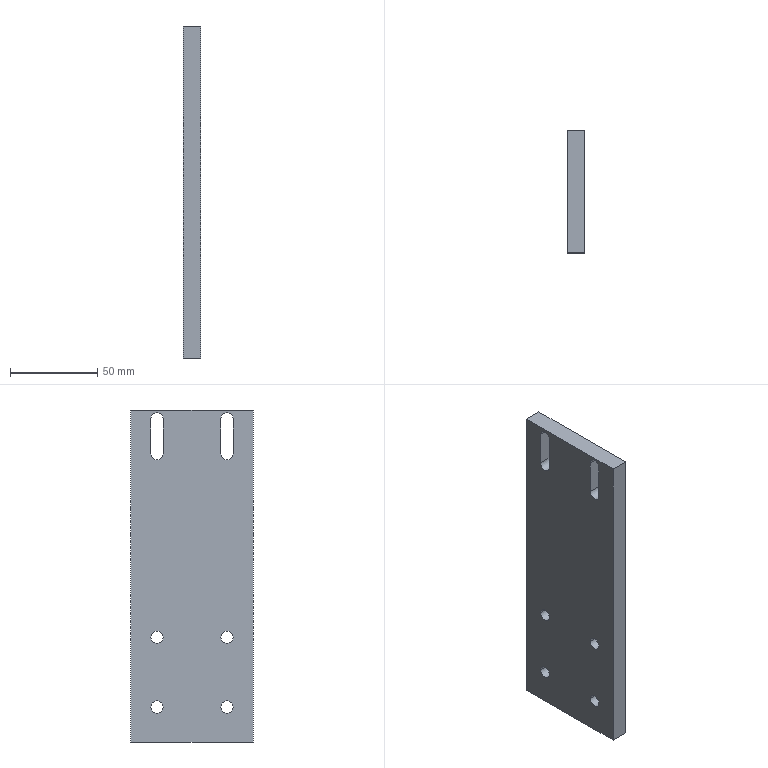Component | SolidWorks | 30-71A-1 | 1 solid | 22 faces | box 10 x 70 x 190 mm | volume 127891 mm3 | cylinder 12 | plane 10 | commonest cylinder face diameters 7 x12
build123d program:
from build123d import *

# Parameters (mm, degrees)
SKETCH1_W          = 70
SKETCH1_H          = 190
EXTRUDE1_DEPTH     = 10
SKETCH8_R          = 3.5
CUT_EXTRUDE1_DEPTH = 102.735
CUT_EXTRUDE2_DEPTH = 10


with BuildPart() as part:
    # Sketch1 → Extrude1 (new body)
    with BuildSketch(Plane.XY):
        Rectangle(SKETCH1_W, SKETCH1_H)
    extrude(amount=EXTRUDE1_DEPTH)

    # Sketch8 → Cut-Extrude1 (cut, through all)
    with BuildSketch(Plane(origin=(0, 0, 0), x_dir=(-1, 0, 0), z_dir=(0, 0, -1))):
        with Locations((-20, -75)):
            Circle(SKETCH8_R)
        with Locations(Location((20, -75, 0), (0, 0, 180))):
            Circle(SKETCH8_R)
        with Locations((20, -35)):
            Circle(SKETCH8_R)
        with Locations(Location((-20, -35, 0), (0, 0, 180))):
            Circle(SKETCH8_R)
    extrude(amount=-CUT_EXTRUDE1_DEPTH, mode=Mode.SUBTRACT)

    # Sketch11 → Cut-Extrude2 (cut)
    with BuildSketch(Plane(origin=(0, 0, 0), x_dir=(-1, 0, 0), z_dir=(0, 0, -1))):
        with BuildLine():
            Line((-23.5, 90), (-23.5, 70))
            ThreePointArc((-23.5, 70), (-20, 66.5), (-16.5, 70))
            Line((-16.5, 70), (-16.5, 90))
            ThreePointArc((-16.5, 90), (-20, 93.5), (-23.5, 90))
        make_face()
        with BuildLine():
            Line((16.5, 70), (16.5, 90))
            ThreePointArc((16.5, 90), (20, 93.5), (23.5, 90))
            Line((23.5, 90), (23.5, 70))
            ThreePointArc((23.5, 70), (20, 66.5), (16.5, 70))
        make_face()
    extrude(amount=-CUT_EXTRUDE2_DEPTH, mode=Mode.SUBTRACT)


solid = part.part

# Placed as in the assembly
solid = solid.moved(Location((302.57, -515.845, 55), (90, -90, 0)))
STEP:
#1=COLOUR_RGB('',0.7922,0.8196,0.9333);
#2=FILL_AREA_STYLE_COLOUR('',#1);
#3=FILL_AREA_STYLE('',(#2));
#4=SURFACE_STYLE_FILL_AREA(#3);
#5=SURFACE_SIDE_STYLE('',(#4));
#6=SURFACE_STYLE_USAGE(.BOTH.,#5);
#7=PRESENTATION_STYLE_ASSIGNMENT((#6));
#8=CARTESIAN_POINT('',(11.519,-21.234,0.7874));
#9=VERTEX_POINT('',#8);
#10=CARTESIAN_POINT('',(11.519,-20.958,0.7874));
#11=VERTEX_POINT('',#10);
#12=CARTESIAN_POINT('',(11.519,-21.096,0.7874));
#13=DIRECTION('',(1.,0.,0.));
#14=DIRECTION('',(0.,-1.,0.));
#15=AXIS2_PLACEMENT_3D('',#12,#13,#14);
#16=CIRCLE('',#15,0.1378);
#17=EDGE_CURVE('',#9,#11,#16,.T.);
#18=ORIENTED_EDGE('',*,*,#17,.F.);
#19=CARTESIAN_POINT('',(11.912,-21.234,0.7874));
#20=VERTEX_POINT('',#19);
#21=CARTESIAN_POINT('',(11.519,-21.234,0.7874));
#22=DIRECTION('',(1.,0.,0.));
#23=VECTOR('',#22,39.37);
#24=LINE('',#21,#23);
#25=EDGE_CURVE('',#9,#20,#24,.T.);
#26=ORIENTED_EDGE('',*,*,#25,.T.);
#27=CARTESIAN_POINT('',(11.912,-20.958,0.7874));
#28=VERTEX_POINT('',#27);
#29=CARTESIAN_POINT('',(11.912,-21.096,0.7874));
#30=DIRECTION('',(1.,0.,0.));
#31=DIRECTION('',(0.,-1.,0.));
#32=AXIS2_PLACEMENT_3D('',#29,#30,#31);
#33=CIRCLE('',#32,0.1378);
#34=EDGE_CURVE('',#20,#28,#33,.T.);
#35=ORIENTED_EDGE('',*,*,#34,.T.);
#36=CARTESIAN_POINT('',(11.519,-20.958,0.7874));
#37=DIRECTION('',(1.,0.,0.));
#38=VECTOR('',#37,39.37);
#39=LINE('',#36,#38);
#40=EDGE_CURVE('',#11,#28,#39,.T.);
#41=ORIENTED_EDGE('',*,*,#40,.F.);
#42=EDGE_LOOP('',(#18,#26,#35,#41));
#43=FACE_OUTER_BOUND('',#42,.T.);
#44=CARTESIAN_POINT('',(11.519,-21.096,0.7874));
#45=DIRECTION('',(1.,0.,0.));
#46=DIRECTION('',(0.,1.,0.));
#47=AXIS2_PLACEMENT_3D('',#44,#45,#46);
#48=CYLINDRICAL_SURFACE('',#47,0.1378);
#49=ADVANCED_FACE('',(#43),#48,.F.);
#50=CARTESIAN_POINT('',(11.519,-19.659,0.7874));
#51=VERTEX_POINT('',#50);
#52=CARTESIAN_POINT('',(11.519,-19.384,0.7874));
#53=VERTEX_POINT('',#52);
#54=CARTESIAN_POINT('',(11.519,-19.521,0.7874));
#55=DIRECTION('',(1.,0.,0.));
#56=DIRECTION('',(0.,1.,0.));
#57=AXIS2_PLACEMENT_3D('',#54,#55,#56);
#58=CIRCLE('',#57,0.1378);
#59=EDGE_CURVE('',#51,#53,#58,.T.);
#60=ORIENTED_EDGE('',*,*,#59,.F.);
#61=CARTESIAN_POINT('',(11.912,-19.659,0.7874));
#62=VERTEX_POINT('',#61);
#63=CARTESIAN_POINT('',(11.519,-19.659,0.7874));
#64=DIRECTION('',(1.,0.,0.));
#65=VECTOR('',#64,39.37);
#66=LINE('',#63,#65);
#67=EDGE_CURVE('',#51,#62,#66,.T.);
#68=ORIENTED_EDGE('',*,*,#67,.T.);
#69=CARTESIAN_POINT('',(11.912,-19.384,0.7874));
#70=VERTEX_POINT('',#69);
#71=CARTESIAN_POINT('',(11.912,-19.521,0.7874));
#72=DIRECTION('',(1.,0.,0.));
#73=DIRECTION('',(0.,1.,0.));
#74=AXIS2_PLACEMENT_3D('',#71,#72,#73);
#75=CIRCLE('',#74,0.1378);
#76=EDGE_CURVE('',#62,#70,#75,.T.);
#77=ORIENTED_EDGE('',*,*,#76,.T.);
#78=CARTESIAN_POINT('',(11.519,-19.384,0.7874));
#79=DIRECTION('',(1.,0.,0.));
#80=VECTOR('',#79,39.37);
#81=LINE('',#78,#80);
#82=EDGE_CURVE('',#53,#70,#81,.T.);
#83=ORIENTED_EDGE('',*,*,#82,.F.);
#84=EDGE_LOOP('',(#60,#68,#77,#83));
#85=FACE_OUTER_BOUND('',#84,.T.);
#86=CARTESIAN_POINT('',(11.519,-19.521,0.7874));
#87=DIRECTION('',(1.,0.,0.));
#88=DIRECTION('',(0.,1.,0.));
#89=AXIS2_PLACEMENT_3D('',#86,#87,#88);
#90=CYLINDRICAL_SURFACE('',#89,0.1378);
#91=ADVANCED_FACE('',(#85),#90,.F.);
#92=CARTESIAN_POINT('',(11.519,-19.659,-0.7874));
#93=VERTEX_POINT('',#92);
#94=CARTESIAN_POINT('',(11.519,-19.384,-0.7874));
#95=VERTEX_POINT('',#94);
#96=CARTESIAN_POINT('',(11.519,-19.521,-0.7874));
#97=DIRECTION('',(1.,0.,0.));
#98=DIRECTION('',(0.,-1.,0.));
#99=AXIS2_PLACEMENT_3D('',#96,#97,#98);
#100=CIRCLE('',#99,0.1378);
#101=EDGE_CURVE('',#93,#95,#100,.T.);
#102=ORIENTED_EDGE('',*,*,#101,.F.);
#103=CARTESIAN_POINT('',(11.912,-19.659,-0.7874));
#104=VERTEX_POINT('',#103);
#105=CARTESIAN_POINT('',(11.519,-19.659,-0.7874));
#106=DIRECTION('',(1.,0.,0.));
#107=VECTOR('',#106,39.37);
#108=LINE('',#105,#107);
#109=EDGE_CURVE('',#93,#104,#108,.T.);
#110=ORIENTED_EDGE('',*,*,#109,.T.);
#111=CARTESIAN_POINT('',(11.912,-19.384,-0.7874));
#112=VERTEX_POINT('',#111);
#113=CARTESIAN_POINT('',(11.912,-19.521,-0.7874));
#114=DIRECTION('',(1.,0.,0.));
#115=DIRECTION('',(0.,-1.,0.));
#116=AXIS2_PLACEMENT_3D('',#113,#114,#115);
#117=CIRCLE('',#116,0.1378);
#118=EDGE_CURVE('',#104,#112,#117,.T.);
#119=ORIENTED_EDGE('',*,*,#118,.T.);
#120=CARTESIAN_POINT('',(11.519,-19.384,-0.7874));
#121=DIRECTION('',(1.,0.,0.));
#122=VECTOR('',#121,39.37);
#123=LINE('',#120,#122);
#124=EDGE_CURVE('',#95,#112,#123,.T.);
#125=ORIENTED_EDGE('',*,*,#124,.F.);
#126=EDGE_LOOP('',(#102,#110,#119,#125));
#127=FACE_OUTER_BOUND('',#126,.T.);
#128=CARTESIAN_POINT('',(11.519,-19.521,-0.7874));
#129=DIRECTION('',(1.,0.,0.));
#130=DIRECTION('',(0.,1.,0.));
#131=AXIS2_PLACEMENT_3D('',#128,#129,#130);
#132=CYLINDRICAL_SURFACE('',#131,0.1378);
#133=ADVANCED_FACE('',(#127),#132,.F.);
#134=CARTESIAN_POINT('',(11.519,-21.234,-0.7874));
#135=VERTEX_POINT('',#134);
#136=CARTESIAN_POINT('',(11.519,-20.958,-0.7874));
#137=VERTEX_POINT('',#136);
#138=CARTESIAN_POINT('',(11.519,-21.096,-0.7874));
#139=DIRECTION('',(1.,0.,0.));
#140=DIRECTION('',(0.,1.,0.));
#141=AXIS2_PLACEMENT_3D('',#138,#139,#140);
#142=CIRCLE('',#141,0.1378);
#143=EDGE_CURVE('',#135,#137,#142,.T.);
#144=ORIENTED_EDGE('',*,*,#143,.F.);
#145=CARTESIAN_POINT('',(11.912,-21.234,-0.7874));
#146=VERTEX_POINT('',#145);
#147=CARTESIAN_POINT('',(11.519,-21.234,-0.7874));
#148=DIRECTION('',(1.,0.,0.));
#149=VECTOR('',#148,39.37);
#150=LINE('',#147,#149);
#151=EDGE_CURVE('',#135,#146,#150,.T.);
#152=ORIENTED_EDGE('',*,*,#151,.T.);
#153=CARTESIAN_POINT('',(11.912,-20.958,-0.7874));
#154=VERTEX_POINT('',#153);
#155=CARTESIAN_POINT('',(11.912,-21.096,-0.7874));
#156=DIRECTION('',(1.,0.,0.));
#157=DIRECTION('',(0.,1.,0.));
#158=AXIS2_PLACEMENT_3D('',#155,#156,#157);
#159=CIRCLE('',#158,0.1378);
#160=EDGE_CURVE('',#146,#154,#159,.T.);
#161=ORIENTED_EDGE('',*,*,#160,.T.);
#162=CARTESIAN_POINT('',(11.519,-20.958,-0.7874));
#163=DIRECTION('',(1.,0.,0.));
#164=VECTOR('',#163,39.37);
#165=LINE('',#162,#164);
#166=EDGE_CURVE('',#137,#154,#165,.T.);
#167=ORIENTED_EDGE('',*,*,#166,.F.);
#168=EDGE_LOOP('',(#144,#152,#161,#167));
#169=FACE_OUTER_BOUND('',#168,.T.);
#170=CARTESIAN_POINT('',(11.519,-21.096,-0.7874));
#171=DIRECTION('',(1.,0.,0.));
#172=DIRECTION('',(0.,1.,0.));
#173=AXIS2_PLACEMENT_3D('',#170,#171,#172);
#174=CYLINDRICAL_SURFACE('',#173,0.1378);
#175=ADVANCED_FACE('',(#169),#174,.F.);
#176=CARTESIAN_POINT('',(11.912,-18.931,5.906));
#177=VERTEX_POINT('',#176);
#178=CARTESIAN_POINT('',(11.912,-18.931,-1.575));
#179=VERTEX_POINT('',#178);
#180=CARTESIAN_POINT('',(11.912,-18.931,5.906));
#181=DIRECTION('',(0.,0.,-1.));
#182=VECTOR('',#181,39.37);
#183=LINE('',#180,#182);
#184=EDGE_CURVE('',#177,#179,#183,.T.);
#185=ORIENTED_EDGE('',*,*,#184,.T.);
#186=CARTESIAN_POINT('',(11.519,-18.931,-1.575));
#187=VERTEX_POINT('',#186);
#188=CARTESIAN_POINT('',(11.519,-18.931,-1.575));
#189=DIRECTION('',(1.,0.,0.));
#190=VECTOR('',#189,39.37);
#191=LINE('',#188,#190);
#192=EDGE_CURVE('',#187,#179,#191,.T.);
#193=ORIENTED_EDGE('',*,*,#192,.F.);
#194=CARTESIAN_POINT('',(11.519,-18.931,5.906));
#195=VERTEX_POINT('',#194);
#196=CARTESIAN_POINT('',(11.519,-18.931,5.906));
#197=DIRECTION('',(0.,0.,-1.));
#198=VECTOR('',#197,39.37);
#199=LINE('',#196,#198);
#200=EDGE_CURVE('',#195,#187,#199,.T.);
#201=ORIENTED_EDGE('',*,*,#200,.F.);
#202=CARTESIAN_POINT('',(11.519,-18.931,5.906));
#203=DIRECTION('',(1.,0.,0.));
#204=VECTOR('',#203,39.37);
#205=LINE('',#202,#204);
#206=EDGE_CURVE('',#195,#177,#205,.T.);
#207=ORIENTED_EDGE('',*,*,#206,.T.);
#208=EDGE_LOOP('',(#185,#193,#201,#207));
#209=FACE_OUTER_BOUND('',#208,.T.);
#210=CARTESIAN_POINT('',(11.519,-18.931,5.906));
#211=DIRECTION('',(0.,-1.,0.));
#212=DIRECTION('',(1.,0.,0.));
#213=AXIS2_PLACEMENT_3D('',#210,#211,#212);
#214=PLANE('',#213);
#215=ADVANCED_FACE('',(#209),#214,.F.);
#216=CARTESIAN_POINT('',(11.912,-21.687,-1.575));
#217=VERTEX_POINT('',#216);
#218=CARTESIAN_POINT('',(11.912,-18.931,-1.575));
#219=DIRECTION('',(-0.,-1.,0.));
#220=VECTOR('',#219,39.37);
#221=LINE('',#218,#220);
#222=EDGE_CURVE('',#179,#217,#221,.T.);
#223=ORIENTED_EDGE('',*,*,#222,.T.);
#224=CARTESIAN_POINT('',(11.519,-21.687,-1.575));
#225=VERTEX_POINT('',#224);
#226=CARTESIAN_POINT('',(11.519,-21.687,-1.575));
#227=DIRECTION('',(1.,0.,0.));
#228=VECTOR('',#227,39.37);
#229=LINE('',#226,#228);
#230=EDGE_CURVE('',#225,#217,#229,.T.);
#231=ORIENTED_EDGE('',*,*,#230,.F.);
#232=CARTESIAN_POINT('',(11.519,-18.931,-1.575));
#233=DIRECTION('',(-0.,-1.,0.));
#234=VECTOR('',#233,39.37);
#235=LINE('',#232,#234);
#236=EDGE_CURVE('',#187,#225,#235,.T.);
#237=ORIENTED_EDGE('',*,*,#236,.F.);
#238=ORIENTED_EDGE('',*,*,#192,.T.);
#239=EDGE_LOOP('',(#223,#231,#237,#238));
#240=FACE_OUTER_BOUND('',#239,.T.);
#241=CARTESIAN_POINT('',(11.519,-18.931,-1.575));
#242=DIRECTION('',(-0.,0.,1.));
#243=DIRECTION('',(-1.,-0.,-0.));
#244=AXIS2_PLACEMENT_3D('',#241,#242,#243);
#245=PLANE('',#244);
#246=ADVANCED_FACE('',(#240),#245,.F.);
#247=CARTESIAN_POINT('',(11.912,-21.687,5.906));
#248=VERTEX_POINT('',#247);
#249=CARTESIAN_POINT('',(11.912,-21.687,5.906));
#250=DIRECTION('',(-0.,0.,1.));
#251=VECTOR('',#250,39.37);
#252=LINE('',#249,#251);
#253=EDGE_CURVE('',#217,#248,#252,.T.);
#254=ORIENTED_EDGE('',*,*,#253,.T.);
#255=CARTESIAN_POINT('',(11.519,-21.687,5.906));
#256=VERTEX_POINT('',#255);
#257=CARTESIAN_POINT('',(11.519,-21.687,5.906));
#258=DIRECTION('',(1.,0.,0.));
#259=VECTOR('',#258,39.37);
#260=LINE('',#257,#259);
#261=EDGE_CURVE('',#256,#248,#260,.T.);
#262=ORIENTED_EDGE('',*,*,#261,.F.);
#263=CARTESIAN_POINT('',(11.519,-21.687,5.906));
#264=DIRECTION('',(-0.,0.,1.));
#265=VECTOR('',#264,39.37);
#266=LINE('',#263,#265);
#267=EDGE_CURVE('',#225,#256,#266,.T.);
#268=ORIENTED_EDGE('',*,*,#267,.F.);
#269=ORIENTED_EDGE('',*,*,#230,.T.);
#270=EDGE_LOOP('',(#254,#262,#268,#269));
#271=FACE_OUTER_BOUND('',#270,.T.);
#272=CARTESIAN_POINT('',(11.519,-21.687,5.906));
#273=DIRECTION('',(-0.,1.,-0.));
#274=DIRECTION('',(-1.,-0.,-0.));
#275=AXIS2_PLACEMENT_3D('',#272,#273,#274);
#276=PLANE('',#275);
#277=ADVANCED_FACE('',(#271),#276,.F.);
#278=CARTESIAN_POINT('',(11.912,-18.931,5.906));
#279=DIRECTION('',(0.,1.,-0.));
#280=VECTOR('',#279,39.37);
#281=LINE('',#278,#280);
#282=EDGE_CURVE('',#248,#177,#281,.T.);
#283=ORIENTED_EDGE('',*,*,#282,.T.);
#284=ORIENTED_EDGE('',*,*,#206,.F.);
#285=CARTESIAN_POINT('',(11.519,-18.931,5.906));
#286=DIRECTION('',(0.,1.,-0.));
#287=VECTOR('',#286,39.37);
#288=LINE('',#285,#287);
#289=EDGE_CURVE('',#256,#195,#288,.T.);
#290=ORIENTED_EDGE('',*,*,#289,.F.);
#291=ORIENTED_EDGE('',*,*,#261,.T.);
#292=EDGE_LOOP('',(#283,#284,#290,#291));
#293=FACE_OUTER_BOUND('',#292,.T.);
#294=CARTESIAN_POINT('',(11.519,-18.931,5.906));
#295=DIRECTION('',(0.,-0.,-1.));
#296=DIRECTION('',(1.,0.,0.));
#297=AXIS2_PLACEMENT_3D('',#294,#295,#296);
#298=PLANE('',#297);
#299=ADVANCED_FACE('',(#293),#298,.F.);
#300=CARTESIAN_POINT('',(11.519,-20.958,5.709));
#301=VERTEX_POINT('',#300);
#302=CARTESIAN_POINT('',(11.519,-21.234,5.709));
#303=VERTEX_POINT('',#302);
#304=CARTESIAN_POINT('',(11.519,-21.096,5.709));
#305=DIRECTION('',(1.,0.,0.));
#306=DIRECTION('',(0.,1.,0.));
#307=AXIS2_PLACEMENT_3D('',#304,#305,#306);
#308=CIRCLE('',#307,0.1378);
#309=EDGE_CURVE('',#301,#303,#308,.T.);
#310=ORIENTED_EDGE('',*,*,#309,.T.);
#311=CARTESIAN_POINT('',(11.519,-21.234,4.921));
#312=VERTEX_POINT('',#311);
#313=CARTESIAN_POINT('',(11.519,-21.234,5.709));
#314=DIRECTION('',(0.,0.,-1.));
#315=VECTOR('',#314,39.37);
#316=LINE('',#313,#315);
#317=EDGE_CURVE('',#303,#312,#316,.T.);
#318=ORIENTED_EDGE('',*,*,#317,.T.);
#319=CARTESIAN_POINT('',(11.519,-20.958,4.921));
#320=VERTEX_POINT('',#319);
#321=CARTESIAN_POINT('',(11.519,-21.096,4.921));
#322=DIRECTION('',(1.,0.,0.));
#323=DIRECTION('',(0.,1.,0.));
#324=AXIS2_PLACEMENT_3D('',#321,#322,#323);
#325=CIRCLE('',#324,0.1378);
#326=EDGE_CURVE('',#312,#320,#325,.T.);
#327=ORIENTED_EDGE('',*,*,#326,.T.);
#328=CARTESIAN_POINT('',(11.519,-20.958,4.921));
#329=DIRECTION('',(-0.,0.,1.));
#330=VECTOR('',#329,39.37);
#331=LINE('',#328,#330);
#332=EDGE_CURVE('',#320,#301,#331,.T.);
#333=ORIENTED_EDGE('',*,*,#332,.T.);
#334=EDGE_LOOP('',(#310,#318,#327,#333));
#335=FACE_BOUND('',#334,.T.);
#336=CARTESIAN_POINT('',(11.519,-19.659,4.921));
#337=VERTEX_POINT('',#336);
#338=CARTESIAN_POINT('',(11.519,-19.384,4.921));
#339=VERTEX_POINT('',#338);
#340=CARTESIAN_POINT('',(11.519,-19.521,4.921));
#341=DIRECTION('',(1.,0.,0.));
#342=DIRECTION('',(0.,-1.,0.));
#343=AXIS2_PLACEMENT_3D('',#340,#341,#342);
#344=CIRCLE('',#343,0.1378);
#345=EDGE_CURVE('',#337,#339,#344,.T.);
#346=ORIENTED_EDGE('',*,*,#345,.T.);
#347=CARTESIAN_POINT('',(11.519,-19.384,5.709));
#348=VERTEX_POINT('',#347);
#349=CARTESIAN_POINT('',(11.519,-19.384,5.709));
#350=DIRECTION('',(-0.,0.,1.));
#351=VECTOR('',#350,39.37);
#352=LINE('',#349,#351);
#353=EDGE_CURVE('',#339,#348,#352,.T.);
#354=ORIENTED_EDGE('',*,*,#353,.T.);
#355=CARTESIAN_POINT('',(11.519,-19.659,5.709));
#356=VERTEX_POINT('',#355);
#357=CARTESIAN_POINT('',(11.519,-19.521,5.709));
#358=DIRECTION('',(1.,0.,0.));
#359=DIRECTION('',(0.,-1.,0.));
#360=AXIS2_PLACEMENT_3D('',#357,#358,#359);
#361=CIRCLE('',#360,0.1378);
#362=EDGE_CURVE('',#348,#356,#361,.T.);
#363=ORIENTED_EDGE('',*,*,#362,.T.);
#364=CARTESIAN_POINT('',(11.519,-19.659,4.921));
#365=DIRECTION('',(0.,0.,-1.));
#366=VECTOR('',#365,39.37);
#367=LINE('',#364,#366);
#368=EDGE_CURVE('',#356,#337,#367,.T.);
#369=ORIENTED_EDGE('',*,*,#368,.T.);
#370=EDGE_LOOP('',(#346,#354,#363,#369));
#371=FACE_BOUND('',#370,.T.);
#372=CARTESIAN_POINT('',(11.519,-21.096,0.7874));
#373=DIRECTION('',(1.,0.,0.));
#374=DIRECTION('',(0.,-1.,0.));
#375=AXIS2_PLACEMENT_3D('',#372,#373,#374);
#376=CIRCLE('',#375,0.1378);
#377=EDGE_CURVE('',#11,#9,#376,.T.);
#378=ORIENTED_EDGE('',*,*,#377,.T.);
#379=ORIENTED_EDGE('',*,*,#17,.T.);
#380=EDGE_LOOP('',(#378,#379));
#381=FACE_BOUND('',#380,.T.);
#382=CARTESIAN_POINT('',(11.519,-19.521,0.7874));
#383=DIRECTION('',(1.,0.,0.));
#384=DIRECTION('',(0.,1.,0.));
#385=AXIS2_PLACEMENT_3D('',#382,#383,#384);
#386=CIRCLE('',#385,0.1378);
#387=EDGE_CURVE('',#53,#51,#386,.T.);
#388=ORIENTED_EDGE('',*,*,#387,.T.);
#389=ORIENTED_EDGE('',*,*,#59,.T.);
#390=EDGE_LOOP('',(#388,#389));
#391=FACE_BOUND('',#390,.T.);
#392=CARTESIAN_POINT('',(11.519,-19.521,-0.7874));
#393=DIRECTION('',(1.,0.,0.));
#394=DIRECTION('',(0.,-1.,0.));
#395=AXIS2_PLACEMENT_3D('',#392,#393,#394);
#396=CIRCLE('',#395,0.1378);
#397=EDGE_CURVE('',#95,#93,#396,.T.);
#398=ORIENTED_EDGE('',*,*,#397,.T.);
#399=ORIENTED_EDGE('',*,*,#101,.T.);
#400=EDGE_LOOP('',(#398,#399));
#401=FACE_BOUND('',#400,.T.);
#402=CARTESIAN_POINT('',(11.519,-21.096,-0.7874));
#403=DIRECTION('',(1.,0.,0.));
#404=DIRECTION('',(0.,1.,0.));
#405=AXIS2_PLACEMENT_3D('',#402,#403,#404);
#406=CIRCLE('',#405,0.1378);
#407=EDGE_CURVE('',#137,#135,#406,.T.);
#408=ORIENTED_EDGE('',*,*,#407,.T.);
#409=ORIENTED_EDGE('',*,*,#143,.T.);
#410=EDGE_LOOP('',(#408,#409));
#411=FACE_BOUND('',#410,.T.);
#412=ORIENTED_EDGE('',*,*,#200,.T.);
#413=ORIENTED_EDGE('',*,*,#236,.T.);
#414=ORIENTED_EDGE('',*,*,#267,.T.);
#415=ORIENTED_EDGE('',*,*,#289,.T.);
#416=EDGE_LOOP('',(#412,#413,#414,#415));
#417=FACE_OUTER_BOUND('',#416,.T.);
#418=CARTESIAN_POINT('',(11.519,-18.931,-1.575));
#419=DIRECTION('',(-1.,0.,-0.));
#420=DIRECTION('',(-0.,-1.,0.));
#421=AXIS2_PLACEMENT_3D('',#418,#419,#420);
#422=PLANE('',#421);
#423=ADVANCED_FACE('',(#335,#371,#381,#391,#401,#411,#417),#422,.T.);
#424=CARTESIAN_POINT('',(11.912,-21.234,5.709));
#425=VERTEX_POINT('',#424);
#426=CARTESIAN_POINT('',(11.912,-21.234,4.921));
#427=VERTEX_POINT('',#426);
#428=CARTESIAN_POINT('',(11.912,-21.234,5.709));
#429=DIRECTION('',(0.,0.,-1.));
#430=VECTOR('',#429,39.37);
#431=LINE('',#428,#430);
#432=EDGE_CURVE('',#425,#427,#431,.T.);
#433=ORIENTED_EDGE('',*,*,#432,.F.);
#434=CARTESIAN_POINT('',(11.912,-20.958,5.709));
#435=VERTEX_POINT('',#434);
#436=CARTESIAN_POINT('',(11.912,-21.096,5.709));
#437=DIRECTION('',(1.,0.,0.));
#438=DIRECTION('',(0.,1.,0.));
#439=AXIS2_PLACEMENT_3D('',#436,#437,#438);
#440=CIRCLE('',#439,0.1378);
#441=EDGE_CURVE('',#435,#425,#440,.T.);
#442=ORIENTED_EDGE('',*,*,#441,.F.);
#443=CARTESIAN_POINT('',(11.912,-20.958,4.921));
#444=VERTEX_POINT('',#443);
#445=CARTESIAN_POINT('',(11.912,-20.958,4.921));
#446=DIRECTION('',(-0.,0.,1.));
#447=VECTOR('',#446,39.37);
#448=LINE('',#445,#447);
#449=EDGE_CURVE('',#444,#435,#448,.T.);
#450=ORIENTED_EDGE('',*,*,#449,.F.);
#451=CARTESIAN_POINT('',(11.912,-21.096,4.921));
#452=DIRECTION('',(1.,0.,0.));
#453=DIRECTION('',(0.,1.,0.));
#454=AXIS2_PLACEMENT_3D('',#451,#452,#453);
#455=CIRCLE('',#454,0.1378);
#456=EDGE_CURVE('',#427,#444,#455,.T.);
#457=ORIENTED_EDGE('',*,*,#456,.F.);
#458=EDGE_LOOP('',(#433,#442,#450,#457));
#459=FACE_BOUND('',#458,.T.);
#460=CARTESIAN_POINT('',(11.912,-19.384,4.921));
#461=VERTEX_POINT('',#460);
#462=CARTESIAN_POINT('',(11.912,-19.384,5.709));
#463=VERTEX_POINT('',#462);
#464=CARTESIAN_POINT('',(11.912,-19.384,5.709));
#465=DIRECTION('',(-0.,0.,1.));
#466=VECTOR('',#465,39.37);
#467=LINE('',#464,#466);
#468=EDGE_CURVE('',#461,#463,#467,.T.);
#469=ORIENTED_EDGE('',*,*,#468,.F.);
#470=CARTESIAN_POINT('',(11.912,-19.659,4.921));
#471=VERTEX_POINT('',#470);
#472=CARTESIAN_POINT('',(11.912,-19.521,4.921));
#473=DIRECTION('',(1.,0.,0.));
#474=DIRECTION('',(0.,-1.,0.));
#475=AXIS2_PLACEMENT_3D('',#472,#473,#474);
#476=CIRCLE('',#475,0.1378);
#477=EDGE_CURVE('',#471,#461,#476,.T.);
#478=ORIENTED_EDGE('',*,*,#477,.F.);
#479=CARTESIAN_POINT('',(11.912,-19.659,5.709));
#480=VERTEX_POINT('',#479);
#481=CARTESIAN_POINT('',(11.912,-19.659,4.921));
#482=DIRECTION('',(0.,0.,-1.));
#483=VECTOR('',#482,39.37);
#484=LINE('',#481,#483);
#485=EDGE_CURVE('',#480,#471,#484,.T.);
#486=ORIENTED_EDGE('',*,*,#485,.F.);
#487=CARTESIAN_POINT('',(11.912,-19.521,5.709));
#488=DIRECTION('',(1.,0.,0.));
#489=DIRECTION('',(0.,-1.,0.));
#490=AXIS2_PLACEMENT_3D('',#487,#488,#489);
#491=CIRCLE('',#490,0.1378);
#492=EDGE_CURVE('',#463,#480,#491,.T.);
#493=ORIENTED_EDGE('',*,*,#492,.F.);
#494=EDGE_LOOP('',(#469,#478,#486,#493));
#495=FACE_BOUND('',#494,.T.);
#496=CARTESIAN_POINT('',(11.912,-21.096,0.7874));
#497=DIRECTION('',(1.,0.,0.));
#498=DIRECTION('',(0.,-1.,0.));
#499=AXIS2_PLACEMENT_3D('',#496,#497,#498);
#500=CIRCLE('',#499,0.1378);
#501=EDGE_CURVE('',#28,#20,#500,.T.);
#502=ORIENTED_EDGE('',*,*,#501,.F.);
#503=ORIENTED_EDGE('',*,*,#34,.F.);
#504=EDGE_LOOP('',(#502,#503));
#505=FACE_BOUND('',#504,.T.);
#506=CARTESIAN_POINT('',(11.912,-19.521,0.7874));
#507=DIRECTION('',(1.,0.,0.));
#508=DIRECTION('',(0.,1.,0.));
#509=AXIS2_PLACEMENT_3D('',#506,#507,#508);
#510=CIRCLE('',#509,0.1378);
#511=EDGE_CURVE('',#70,#62,#510,.T.);
#512=ORIENTED_EDGE('',*,*,#511,.F.);
#513=ORIENTED_EDGE('',*,*,#76,.F.);
#514=EDGE_LOOP('',(#512,#513));
#515=FACE_BOUND('',#514,.T.);
#516=CARTESIAN_POINT('',(11.912,-19.521,-0.7874));
#517=DIRECTION('',(1.,0.,0.));
#518=DIRECTION('',(0.,-1.,0.));
#519=AXIS2_PLACEMENT_3D('',#516,#517,#518);
#520=CIRCLE('',#519,0.1378);
#521=EDGE_CURVE('',#112,#104,#520,.T.);
#522=ORIENTED_EDGE('',*,*,#521,.F.);
#523=ORIENTED_EDGE('',*,*,#118,.F.);
#524=EDGE_LOOP('',(#522,#523));
#525=FACE_BOUND('',#524,.T.);
#526=CARTESIAN_POINT('',(11.912,-21.096,-0.7874));
#527=DIRECTION('',(1.,0.,0.));
#528=DIRECTION('',(0.,1.,0.));
#529=AXIS2_PLACEMENT_3D('',#526,#527,#528);
#530=CIRCLE('',#529,0.1378);
#531=EDGE_CURVE('',#154,#146,#530,.T.);
#532=ORIENTED_EDGE('',*,*,#531,.F.);
#533=ORIENTED_EDGE('',*,*,#160,.F.);
#534=EDGE_LOOP('',(#532,#533));
#535=FACE_BOUND('',#534,.T.);
#536=ORIENTED_EDGE('',*,*,#184,.F.);
#537=ORIENTED_EDGE('',*,*,#282,.F.);
#538=ORIENTED_EDGE('',*,*,#253,.F.);
#539=ORIENTED_EDGE('',*,*,#222,.F.);
#540=EDGE_LOOP('',(#536,#537,#538,#539));
#541=FACE_OUTER_BOUND('',#540,.T.);
#542=CARTESIAN_POINT('',(11.912,-18.931,-1.575));
#543=DIRECTION('',(-1.,0.,-0.));
#544=DIRECTION('',(-0.,-1.,0.));
#545=AXIS2_PLACEMENT_3D('',#542,#543,#544);
#546=PLANE('',#545);
#547=ADVANCED_FACE('',(#459,#495,#505,#515,#525,#535,#541),#546,.F.);
#548=ORIENTED_EDGE('',*,*,#151,.F.);
#549=ORIENTED_EDGE('',*,*,#407,.F.);
#550=ORIENTED_EDGE('',*,*,#166,.T.);
#551=ORIENTED_EDGE('',*,*,#531,.T.);
#552=EDGE_LOOP('',(#548,#549,#550,#551));
#553=FACE_OUTER_BOUND('',#552,.T.);
#554=CARTESIAN_POINT('',(11.519,-21.096,-0.7874));
#555=DIRECTION('',(1.,0.,0.));
#556=DIRECTION('',(0.,1.,0.));
#557=AXIS2_PLACEMENT_3D('',#554,#555,#556);
#558=CYLINDRICAL_SURFACE('',#557,0.1378);
#559=ADVANCED_FACE('',(#553),#558,.F.);
#560=ORIENTED_EDGE('',*,*,#109,.F.);
#561=ORIENTED_EDGE('',*,*,#397,.F.);
#562=ORIENTED_EDGE('',*,*,#124,.T.);
#563=ORIENTED_EDGE('',*,*,#521,.T.);
#564=EDGE_LOOP('',(#560,#561,#562,#563));
#565=FACE_OUTER_BOUND('',#564,.T.);
#566=CARTESIAN_POINT('',(11.519,-19.521,-0.7874));
#567=DIRECTION('',(1.,0.,0.));
#568=DIRECTION('',(0.,1.,0.));
#569=AXIS2_PLACEMENT_3D('',#566,#567,#568);
#570=CYLINDRICAL_SURFACE('',#569,0.1378);
#571=ADVANCED_FACE('',(#565),#570,.F.);
#572=ORIENTED_EDGE('',*,*,#67,.F.);
#573=ORIENTED_EDGE('',*,*,#387,.F.);
#574=ORIENTED_EDGE('',*,*,#82,.T.);
#575=ORIENTED_EDGE('',*,*,#511,.T.);
#576=EDGE_LOOP('',(#572,#573,#574,#575));
#577=FACE_OUTER_BOUND('',#576,.T.);
#578=CARTESIAN_POINT('',(11.519,-19.521,0.7874));
#579=DIRECTION('',(1.,0.,0.));
#580=DIRECTION('',(0.,1.,0.));
#581=AXIS2_PLACEMENT_3D('',#578,#579,#580);
#582=CYLINDRICAL_SURFACE('',#581,0.1378);
#583=ADVANCED_FACE('',(#577),#582,.F.);
#584=ORIENTED_EDGE('',*,*,#25,.F.);
#585=ORIENTED_EDGE('',*,*,#377,.F.);
#586=ORIENTED_EDGE('',*,*,#40,.T.);
#587=ORIENTED_EDGE('',*,*,#501,.T.);
#588=EDGE_LOOP('',(#584,#585,#586,#587));
#589=FACE_OUTER_BOUND('',#588,.T.);
#590=CARTESIAN_POINT('',(11.519,-21.096,0.7874));
#591=DIRECTION('',(1.,0.,0.));
#592=DIRECTION('',(0.,1.,0.));
#593=AXIS2_PLACEMENT_3D('',#590,#591,#592);
#594=CYLINDRICAL_SURFACE('',#593,0.1378);
#595=ADVANCED_FACE('',(#589),#594,.F.);
#596=ORIENTED_EDGE('',*,*,#477,.T.);
#597=CARTESIAN_POINT('',(11.519,-19.384,4.921));
#598=DIRECTION('',(1.,0.,0.));
#599=VECTOR('',#598,39.37);
#600=LINE('',#597,#599);
#601=EDGE_CURVE('',#339,#461,#600,.T.);
#602=ORIENTED_EDGE('',*,*,#601,.F.);
#603=ORIENTED_EDGE('',*,*,#345,.F.);
#604=CARTESIAN_POINT('',(11.519,-19.659,4.921));
#605=DIRECTION('',(1.,0.,0.));
#606=VECTOR('',#605,39.37);
#607=LINE('',#604,#606);
#608=EDGE_CURVE('',#337,#471,#607,.T.);
#609=ORIENTED_EDGE('',*,*,#608,.T.);
#610=EDGE_LOOP('',(#596,#602,#603,#609));
#611=FACE_OUTER_BOUND('',#610,.T.);
#612=CARTESIAN_POINT('',(11.519,-19.521,4.921));
#613=DIRECTION('',(1.,0.,0.));
#614=DIRECTION('',(0.,1.,0.));
#615=AXIS2_PLACEMENT_3D('',#612,#613,#614);
#616=CYLINDRICAL_SURFACE('',#615,0.1378);
#617=ADVANCED_FACE('',(#611),#616,.F.);
#618=ORIENTED_EDGE('',*,*,#485,.T.);
#619=ORIENTED_EDGE('',*,*,#608,.F.);
#620=ORIENTED_EDGE('',*,*,#368,.F.);
#621=CARTESIAN_POINT('',(11.519,-19.659,5.709));
#622=DIRECTION('',(1.,0.,0.));
#623=VECTOR('',#622,39.37);
#624=LINE('',#621,#623);
#625=EDGE_CURVE('',#356,#480,#624,.T.);
#626=ORIENTED_EDGE('',*,*,#625,.T.);
#627=EDGE_LOOP('',(#618,#619,#620,#626));
#628=FACE_OUTER_BOUND('',#627,.T.);
#629=CARTESIAN_POINT('',(11.519,-19.659,4.921));
#630=DIRECTION('',(0.,-1.,0.));
#631=DIRECTION('',(1.,0.,0.));
#632=AXIS2_PLACEMENT_3D('',#629,#630,#631);
#633=PLANE('',#632);
#634=ADVANCED_FACE('',(#628),#633,.F.);
#635=ORIENTED_EDGE('',*,*,#492,.T.);
#636=ORIENTED_EDGE('',*,*,#625,.F.);
#637=ORIENTED_EDGE('',*,*,#362,.F.);
#638=CARTESIAN_POINT('',(11.519,-19.384,5.709));
#639=DIRECTION('',(1.,0.,0.));
#640=VECTOR('',#639,39.37);
#641=LINE('',#638,#640);
#642=EDGE_CURVE('',#348,#463,#641,.T.);
#643=ORIENTED_EDGE('',*,*,#642,.T.);
#644=EDGE_LOOP('',(#635,#636,#637,#643));
#645=FACE_OUTER_BOUND('',#644,.T.);
#646=CARTESIAN_POINT('',(11.519,-19.521,5.709));
#647=DIRECTION('',(1.,0.,0.));
#648=DIRECTION('',(0.,1.,0.));
#649=AXIS2_PLACEMENT_3D('',#646,#647,#648);
#650=CYLINDRICAL_SURFACE('',#649,0.1378);
#651=ADVANCED_FACE('',(#645),#650,.F.);
#652=ORIENTED_EDGE('',*,*,#468,.T.);
#653=ORIENTED_EDGE('',*,*,#642,.F.);
#654=ORIENTED_EDGE('',*,*,#353,.F.);
#655=ORIENTED_EDGE('',*,*,#601,.T.);
#656=EDGE_LOOP('',(#652,#653,#654,#655));
#657=FACE_OUTER_BOUND('',#656,.T.);
#658=CARTESIAN_POINT('',(11.519,-19.384,5.709));
#659=DIRECTION('',(0.,1.,-0.));
#660=DIRECTION('',(0.,-0.,-1.));
#661=AXIS2_PLACEMENT_3D('',#658,#659,#660);
#662=PLANE('',#661);
#663=ADVANCED_FACE('',(#657),#662,.F.);
#664=ORIENTED_EDGE('',*,*,#441,.T.);
#665=CARTESIAN_POINT('',(11.519,-21.234,5.709));
#666=DIRECTION('',(1.,0.,0.));
#667=VECTOR('',#666,39.37);
#668=LINE('',#665,#667);
#669=EDGE_CURVE('',#303,#425,#668,.T.);
#670=ORIENTED_EDGE('',*,*,#669,.F.);
#671=ORIENTED_EDGE('',*,*,#309,.F.);
#672=CARTESIAN_POINT('',(11.519,-20.958,5.709));
#673=DIRECTION('',(1.,0.,0.));
#674=VECTOR('',#673,39.37);
#675=LINE('',#672,#674);
#676=EDGE_CURVE('',#301,#435,#675,.T.);
#677=ORIENTED_EDGE('',*,*,#676,.T.);
#678=EDGE_LOOP('',(#664,#670,#671,#677));
#679=FACE_OUTER_BOUND('',#678,.T.);
#680=CARTESIAN_POINT('',(11.519,-21.096,5.709));
#681=DIRECTION('',(1.,0.,0.));
#682=DIRECTION('',(0.,1.,0.));
#683=AXIS2_PLACEMENT_3D('',#680,#681,#682);
#684=CYLINDRICAL_SURFACE('',#683,0.1378);
#685=ADVANCED_FACE('',(#679),#684,.F.);
#686=ORIENTED_EDGE('',*,*,#449,.T.);
#687=ORIENTED_EDGE('',*,*,#676,.F.);
#688=ORIENTED_EDGE('',*,*,#332,.F.);
#689=CARTESIAN_POINT('',(11.519,-20.958,4.921));
#690=DIRECTION('',(1.,0.,0.));
#691=VECTOR('',#690,39.37);
#692=LINE('',#689,#691);
#693=EDGE_CURVE('',#320,#444,#692,.T.);
#694=ORIENTED_EDGE('',*,*,#693,.T.);
#695=EDGE_LOOP('',(#686,#687,#688,#694));
#696=FACE_OUTER_BOUND('',#695,.T.);
#697=CARTESIAN_POINT('',(11.519,-20.958,4.921));
#698=DIRECTION('',(-0.,1.,-0.));
#699=DIRECTION('',(-1.,-0.,-0.));
#700=AXIS2_PLACEMENT_3D('',#697,#698,#699);
#701=PLANE('',#700);
#702=ADVANCED_FACE('',(#696),#701,.F.);
#703=ORIENTED_EDGE('',*,*,#456,.T.);
#704=ORIENTED_EDGE('',*,*,#693,.F.);
#705=ORIENTED_EDGE('',*,*,#326,.F.);
#706=CARTESIAN_POINT('',(11.519,-21.234,4.921));
#707=DIRECTION('',(1.,0.,0.));
#708=VECTOR('',#707,39.37);
#709=LINE('',#706,#708);
#710=EDGE_CURVE('',#312,#427,#709,.T.);
#711=ORIENTED_EDGE('',*,*,#710,.T.);
#712=EDGE_LOOP('',(#703,#704,#705,#711));
#713=FACE_OUTER_BOUND('',#712,.T.);
#714=CARTESIAN_POINT('',(11.519,-21.096,4.921));
#715=DIRECTION('',(1.,0.,0.));
#716=DIRECTION('',(0.,1.,0.));
#717=AXIS2_PLACEMENT_3D('',#714,#715,#716);
#718=CYLINDRICAL_SURFACE('',#717,0.1378);
#719=ADVANCED_FACE('',(#713),#718,.F.);
#720=ORIENTED_EDGE('',*,*,#432,.T.);
#721=ORIENTED_EDGE('',*,*,#710,.F.);
#722=ORIENTED_EDGE('',*,*,#317,.F.);
#723=ORIENTED_EDGE('',*,*,#669,.T.);
#724=EDGE_LOOP('',(#720,#721,#722,#723));
#725=FACE_OUTER_BOUND('',#724,.T.);
#726=CARTESIAN_POINT('',(11.519,-21.234,5.709));
#727=DIRECTION('',(-0.,-1.,-0.));
#728=DIRECTION('',(-0.,-0.,1.));
#729=AXIS2_PLACEMENT_3D('',#726,#727,#728);
#730=PLANE('',#729);
#731=ADVANCED_FACE('',(#725),#730,.F.);
#732=CLOSED_SHELL('',(#49,#91,#133,#175,#215,#246,#277,#299,#423,#547,#559,#571,#583,#595,#617,#634,#651,#663,#685,#702,#719,#731));
#733=MANIFOLD_SOLID_BREP('',#732);
#734=STYLED_ITEM('',(#7),#733);
#735=(LENGTH_UNIT()NAMED_UNIT(*)SI_UNIT($,.METRE.));
#736=LENGTH_MEASURE_WITH_UNIT(LENGTH_MEASURE(0.0254),#735);
#737=DIMENSIONAL_EXPONENTS(1.,0.,0.,0.,0.,0.,0.);
#738=(CONVERSION_BASED_UNIT('',#736)LENGTH_UNIT()NAMED_UNIT(#737));
#739=UNCERTAINTY_MEASURE_WITH_UNIT(LENGTH_MEASURE(0.00001),#738,'','');
#740=(NAMED_UNIT(*)PLANE_ANGLE_UNIT()SI_UNIT($,.RADIAN.));
#741=(NAMED_UNIT(*)SI_UNIT($,.STERADIAN.)SOLID_ANGLE_UNIT());
#742=(GEOMETRIC_REPRESENTATION_CONTEXT(3)GLOBAL_UNCERTAINTY_ASSIGNED_CONTEXT((#739))GLOBAL_UNIT_ASSIGNED_CONTEXT((#738,#740,#741))REPRESENTATION_CONTEXT('',''));
#743=MECHANICAL_DESIGN_GEOMETRIC_PRESENTATION_REPRESENTATION('',(#734),#742);
#744=PRESENTATION_LAYER_ASSIGNMENT('','',(#734));
#745=CARTESIAN_POINT('',(0.,0.,0.));
#746=DIRECTION('',(0.,0.,1.));
#747=DIRECTION('',(1.,0.,0.));
#748=AXIS2_PLACEMENT_3D('',#745,#746,#747);
#749=(LENGTH_UNIT()NAMED_UNIT(*)SI_UNIT($,.METRE.));
#750=LENGTH_MEASURE_WITH_UNIT(LENGTH_MEASURE(0.0254),#749);
#751=DIMENSIONAL_EXPONENTS(1.,0.,0.,0.,0.,0.,0.);
#752=(CONVERSION_BASED_UNIT('',#750)LENGTH_UNIT()NAMED_UNIT(#751));
#753=UNCERTAINTY_MEASURE_WITH_UNIT(LENGTH_MEASURE(0.00001),#752,'','');
#754=(NAMED_UNIT(*)PLANE_ANGLE_UNIT()SI_UNIT($,.RADIAN.));
#755=(NAMED_UNIT(*)SI_UNIT($,.STERADIAN.)SOLID_ANGLE_UNIT());
#756=(GEOMETRIC_REPRESENTATION_CONTEXT(3)GLOBAL_UNCERTAINTY_ASSIGNED_CONTEXT((#753))GLOBAL_UNIT_ASSIGNED_CONTEXT((#752,#754,#755))REPRESENTATION_CONTEXT('',''));
#757=ADVANCED_BREP_SHAPE_REPRESENTATION('',(#733,#748),#756);